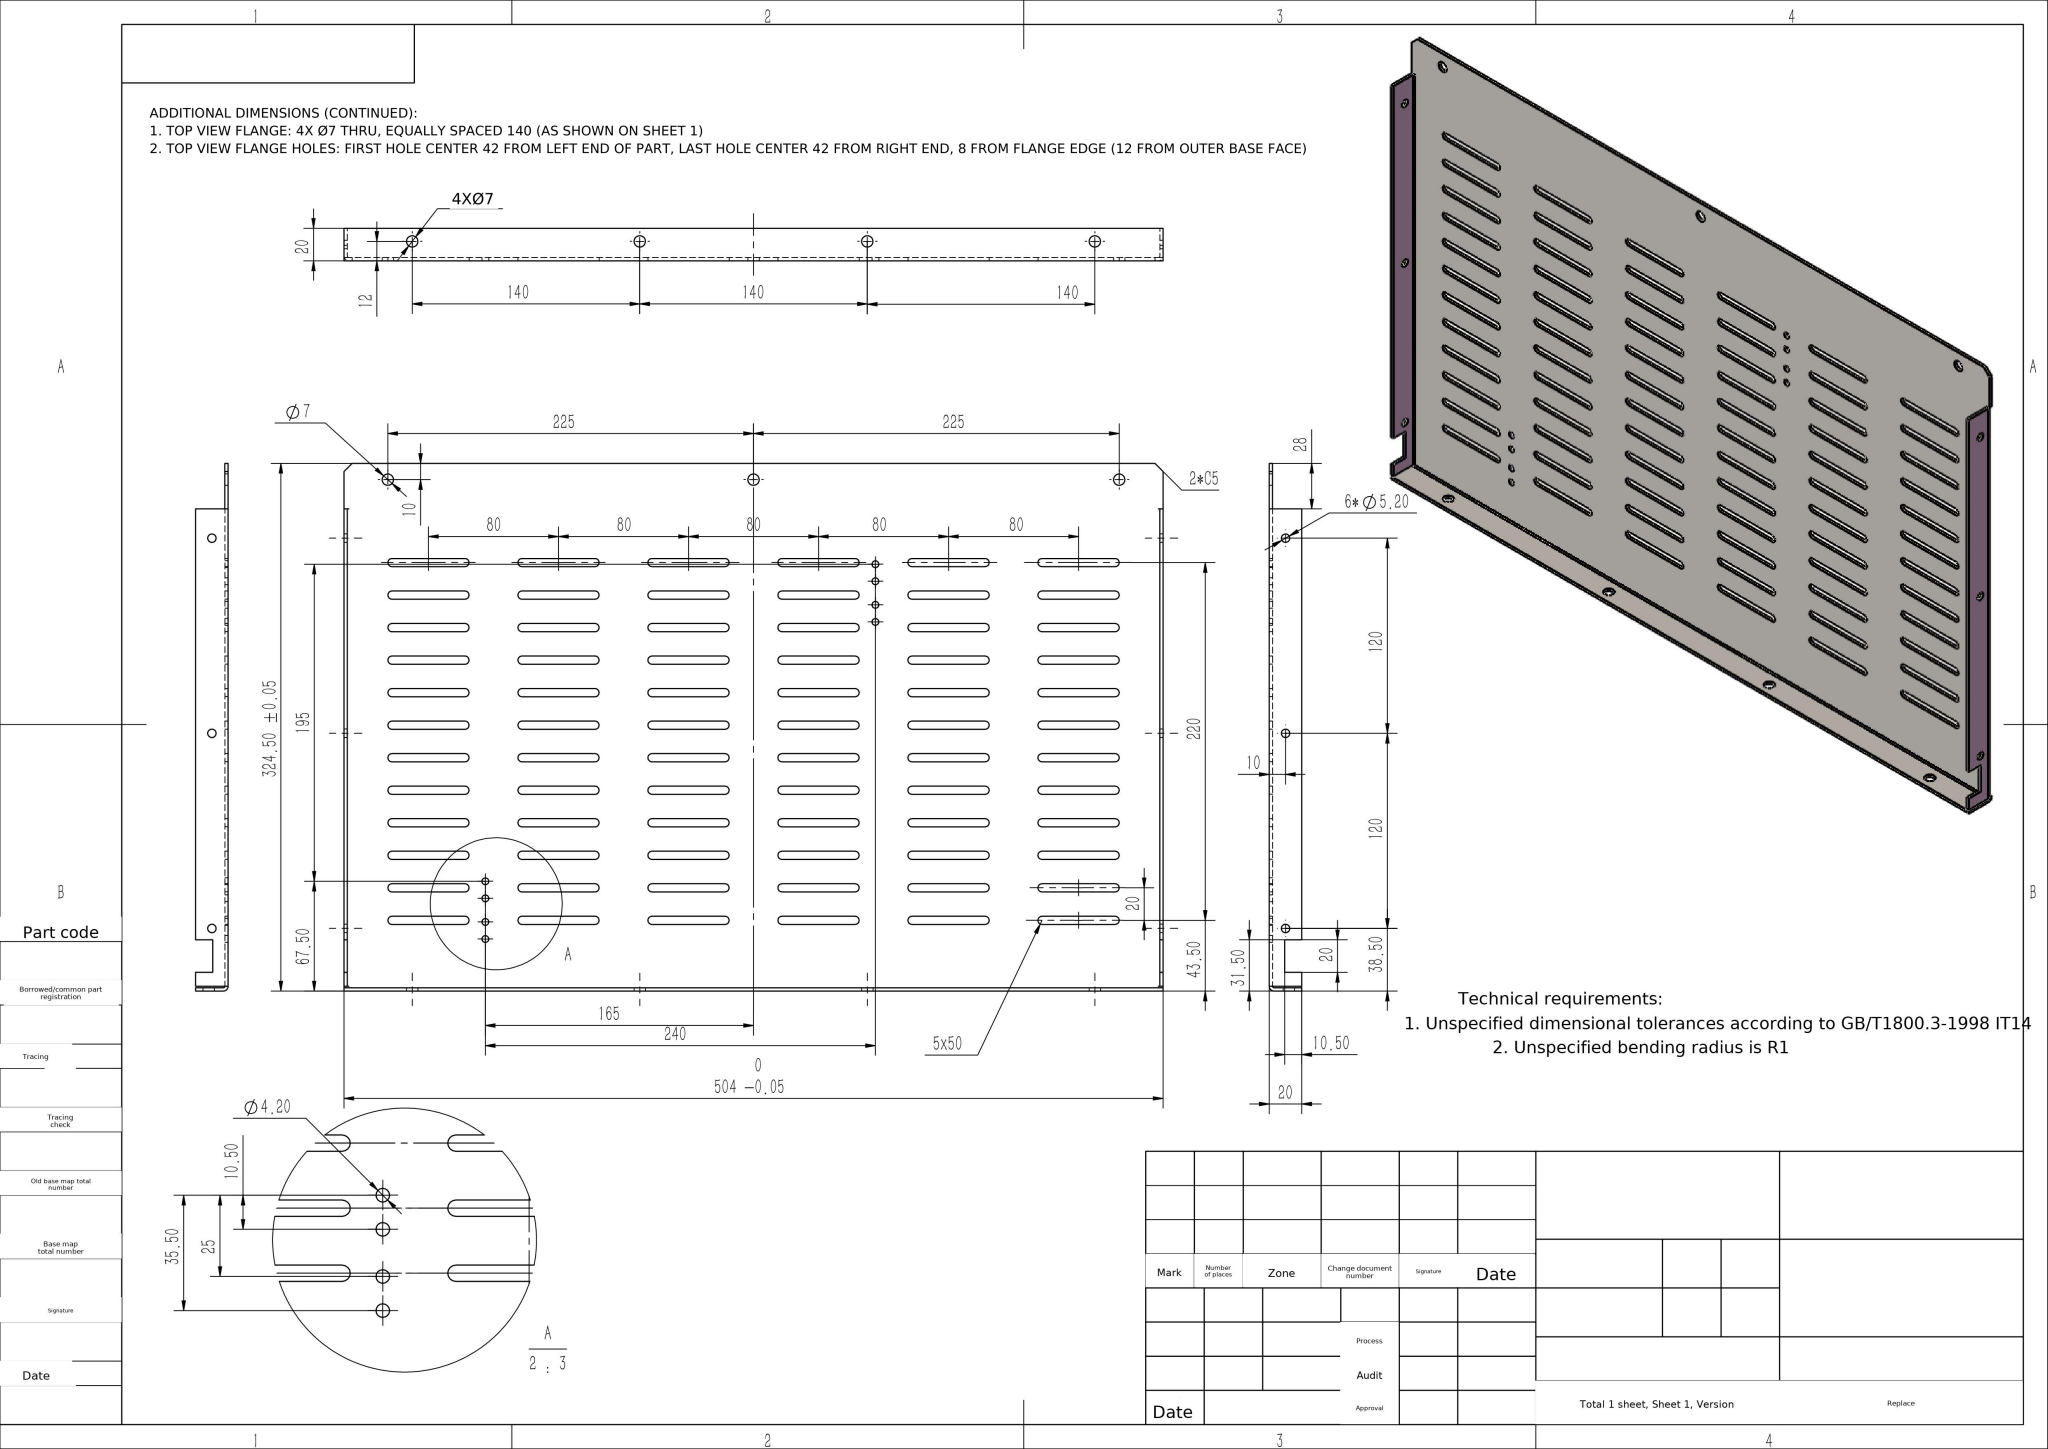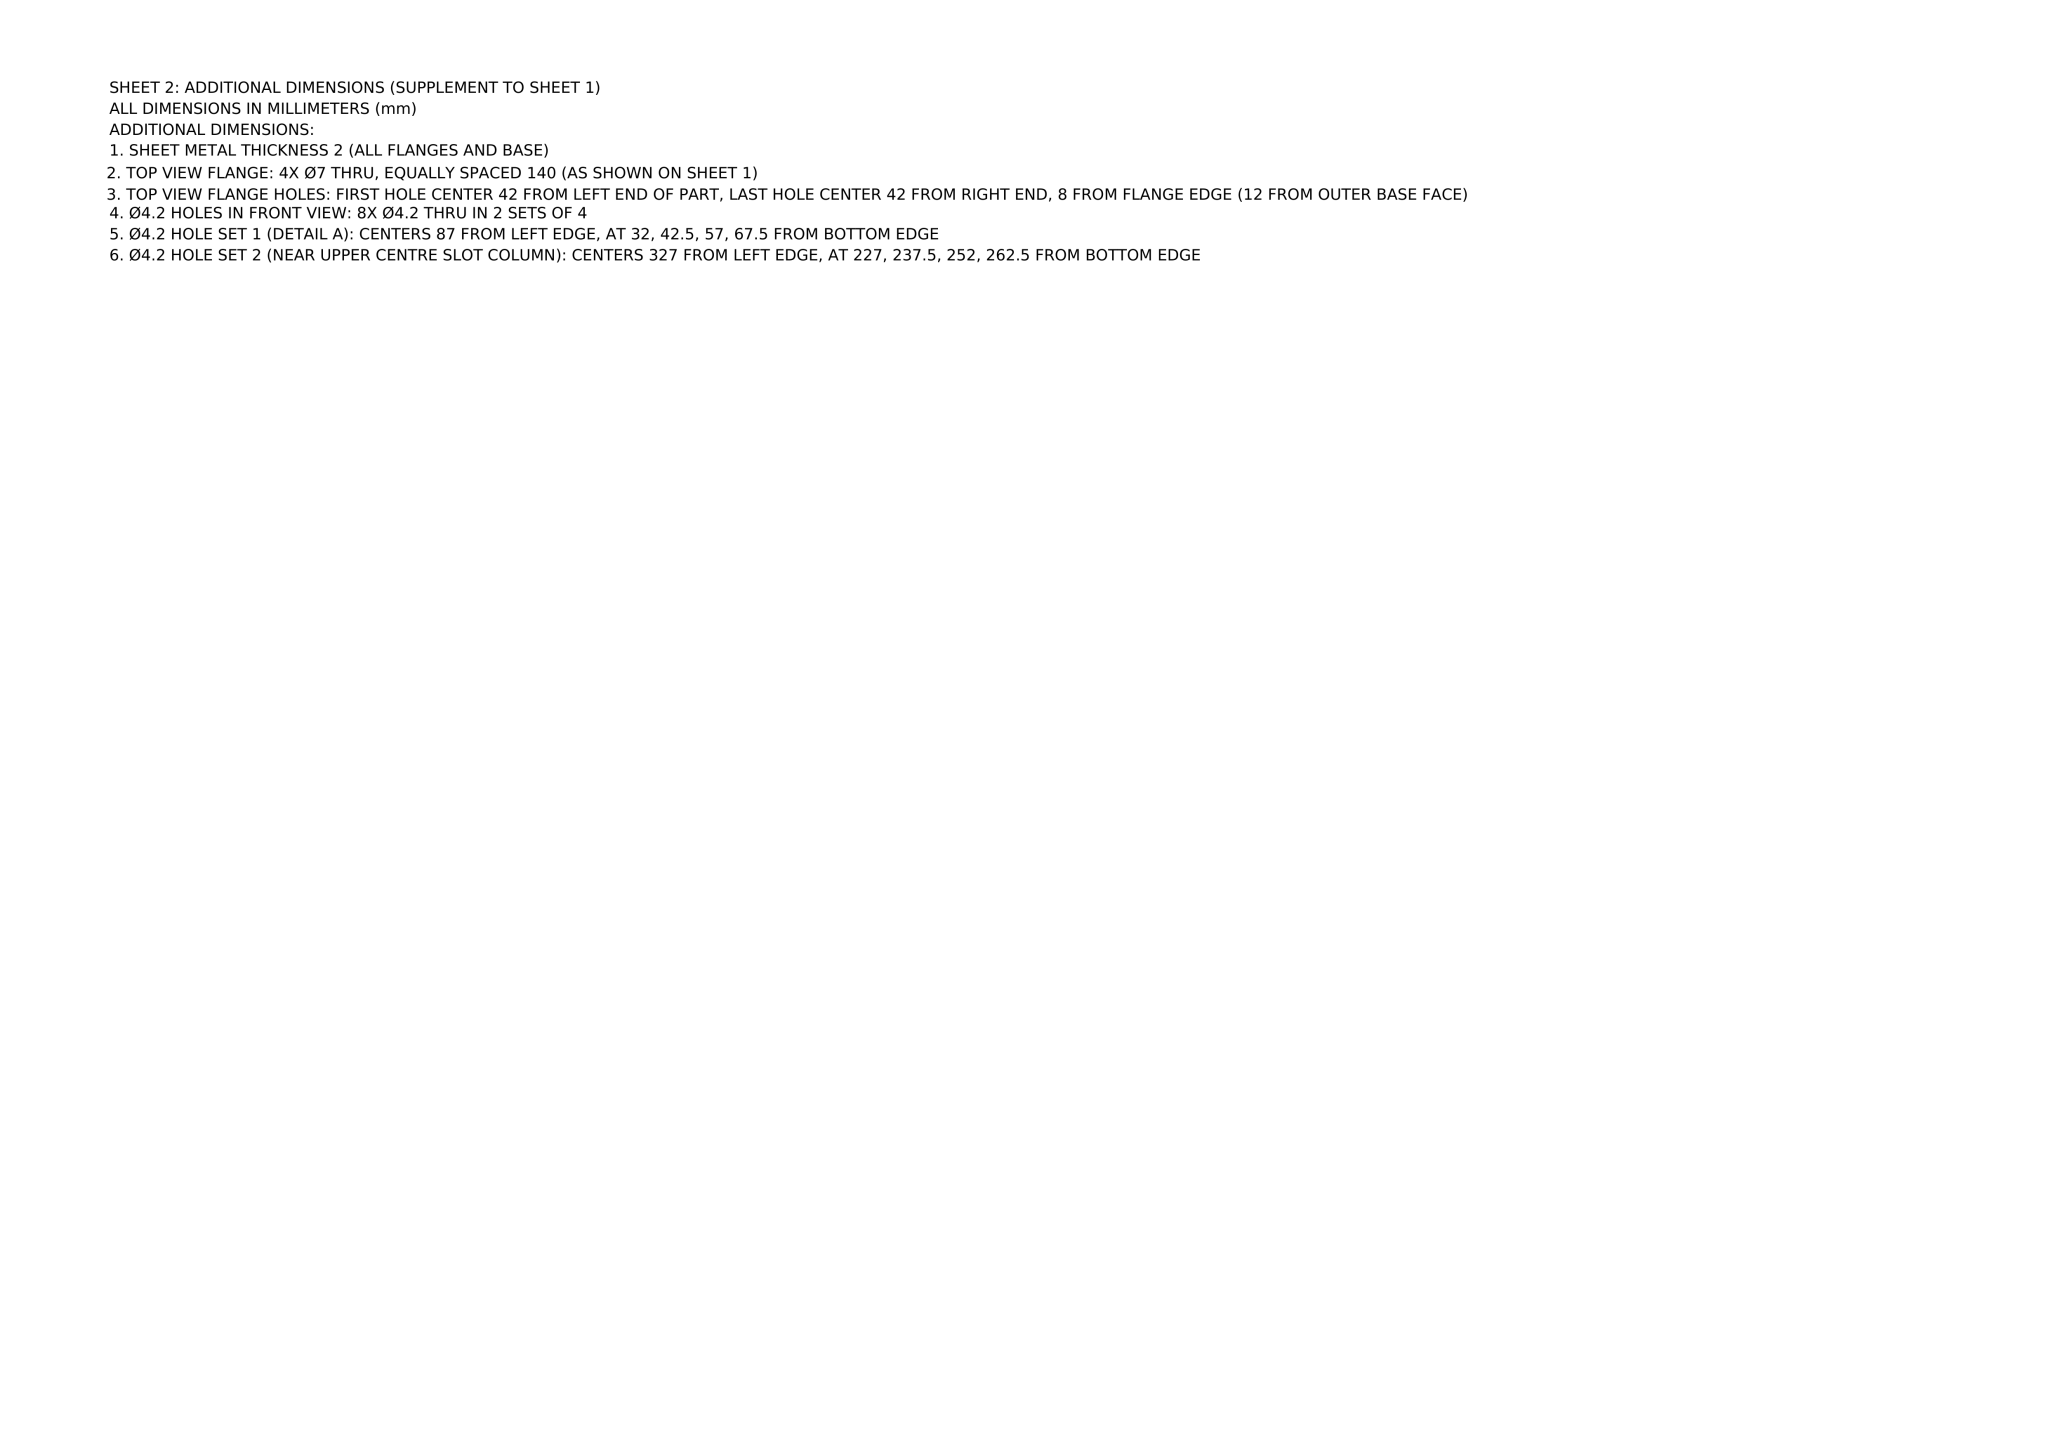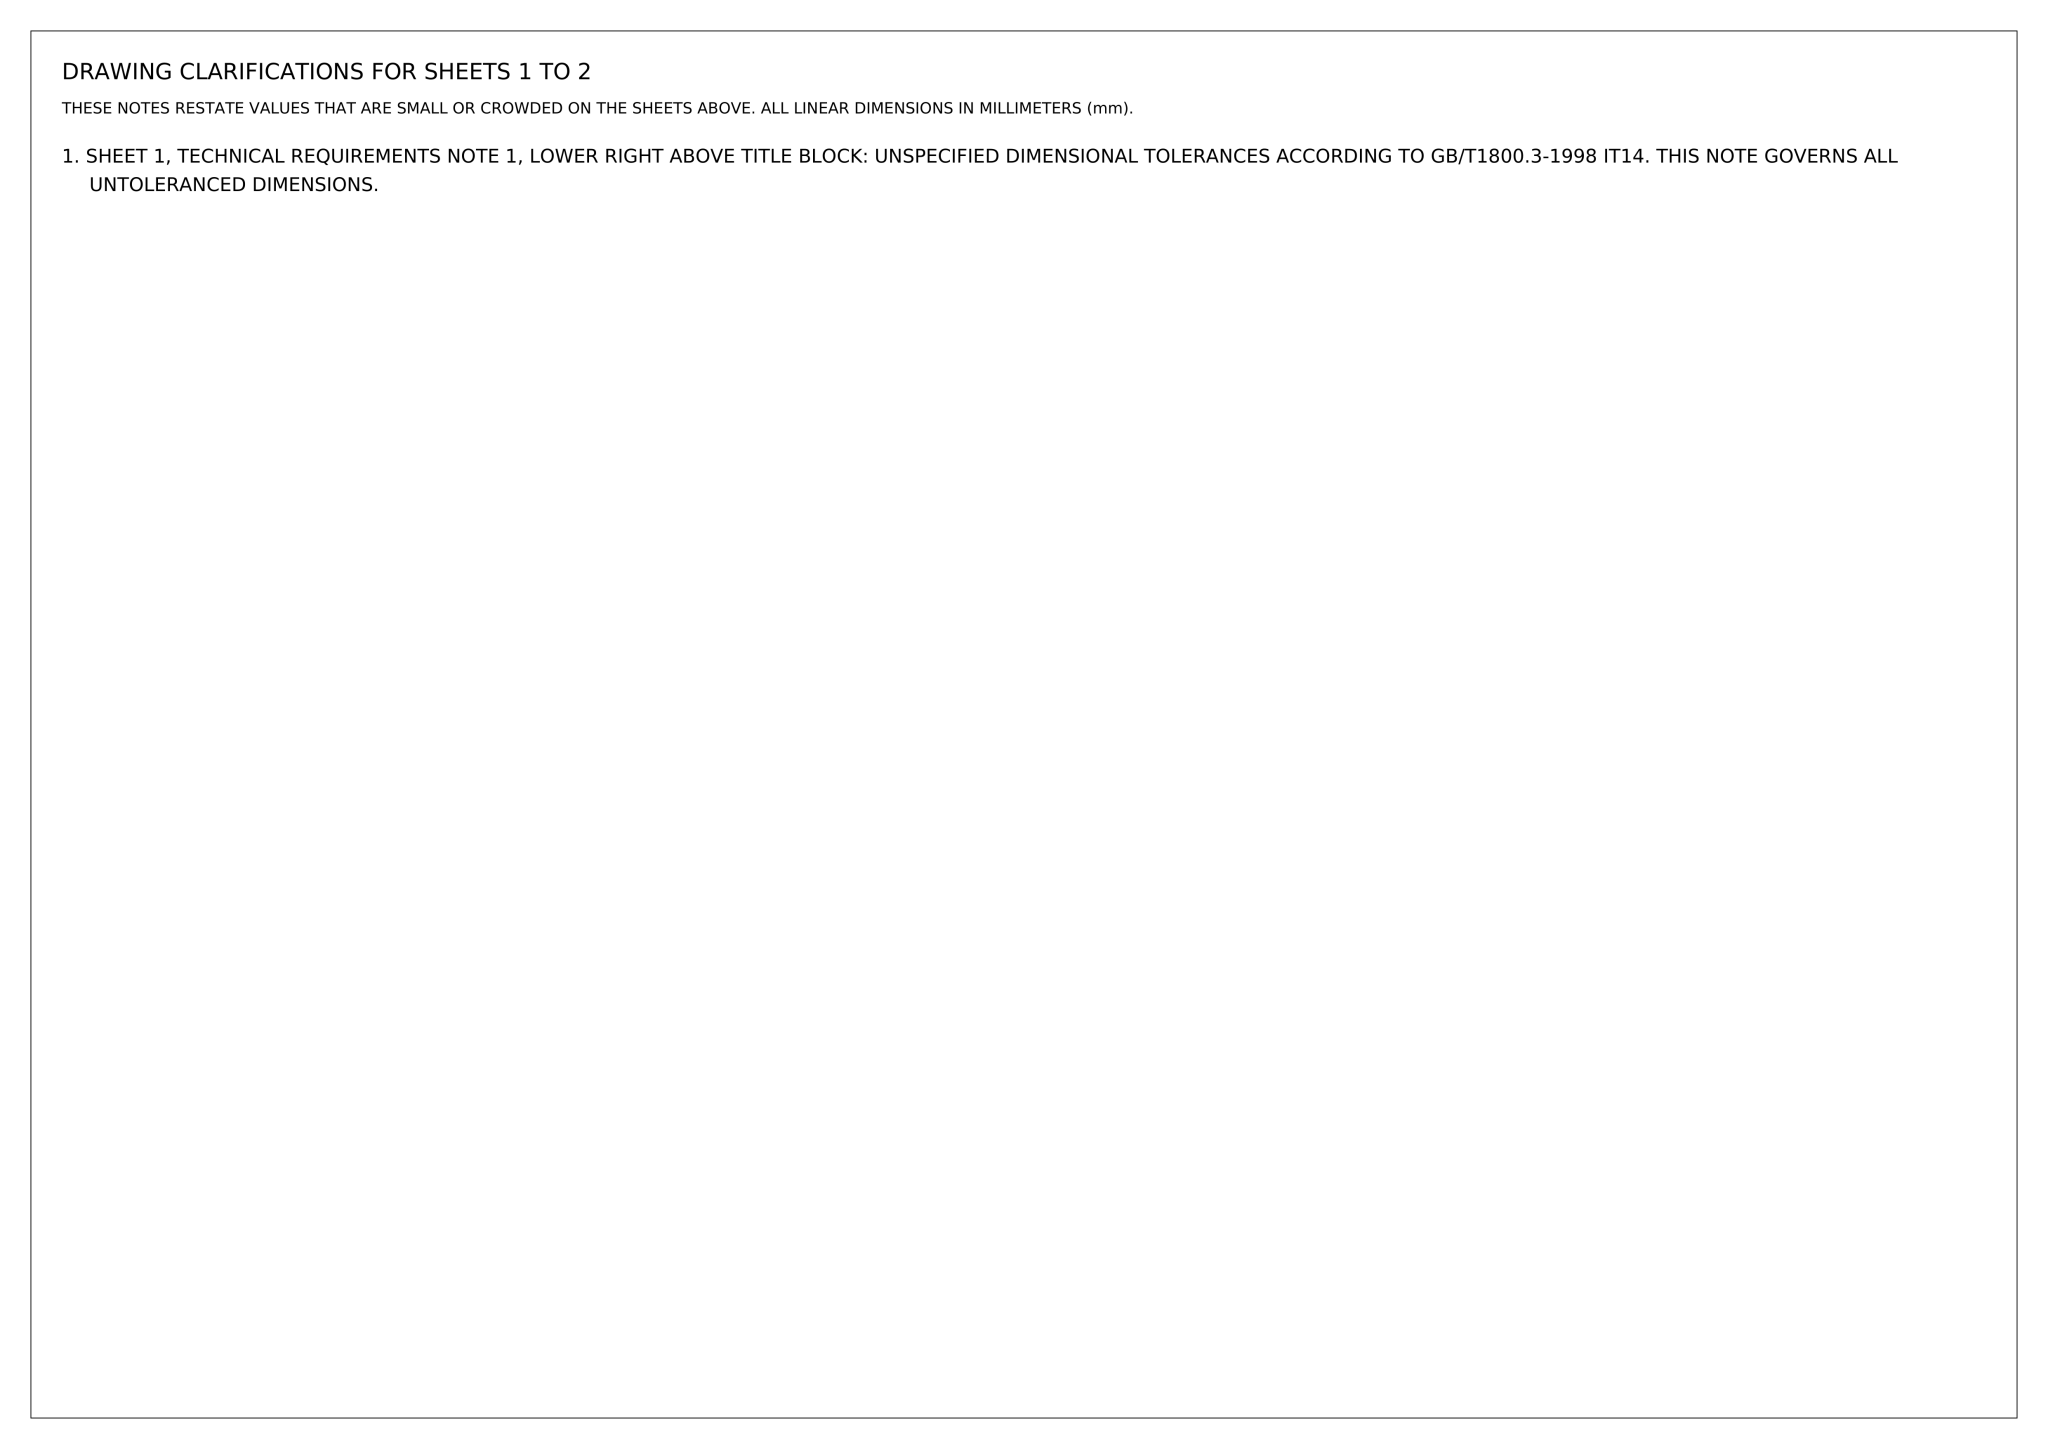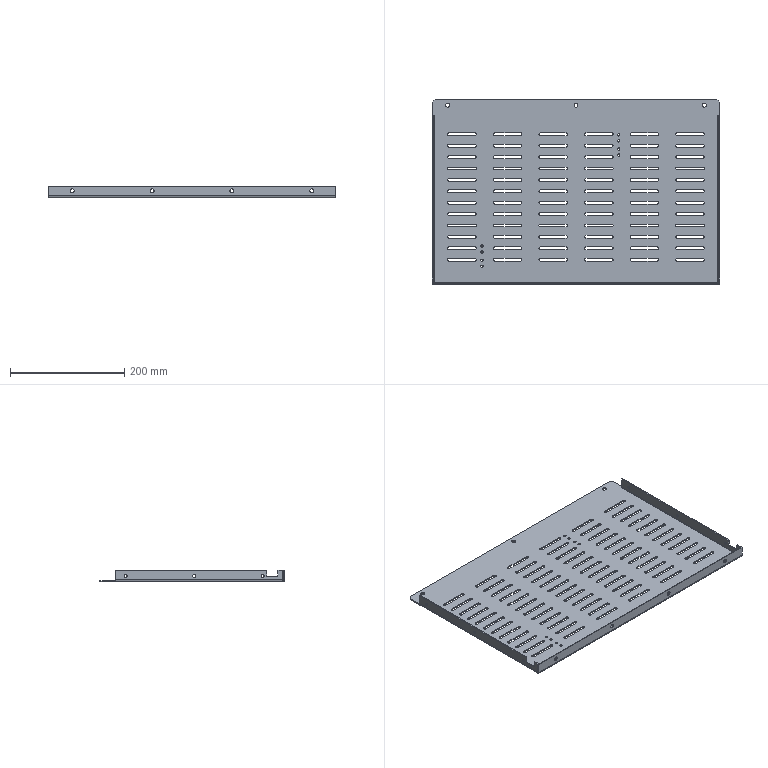Part | NX | mm | 1 solid | 448 faces | box 504 x 324.5 x 20 mm | volume 327366 mm3 | cylinder 264 | plane 184 | commonest cylinder face diameters 5 x216 4.2 x16 7 x14 5.2 x12 6 x3 2 x3